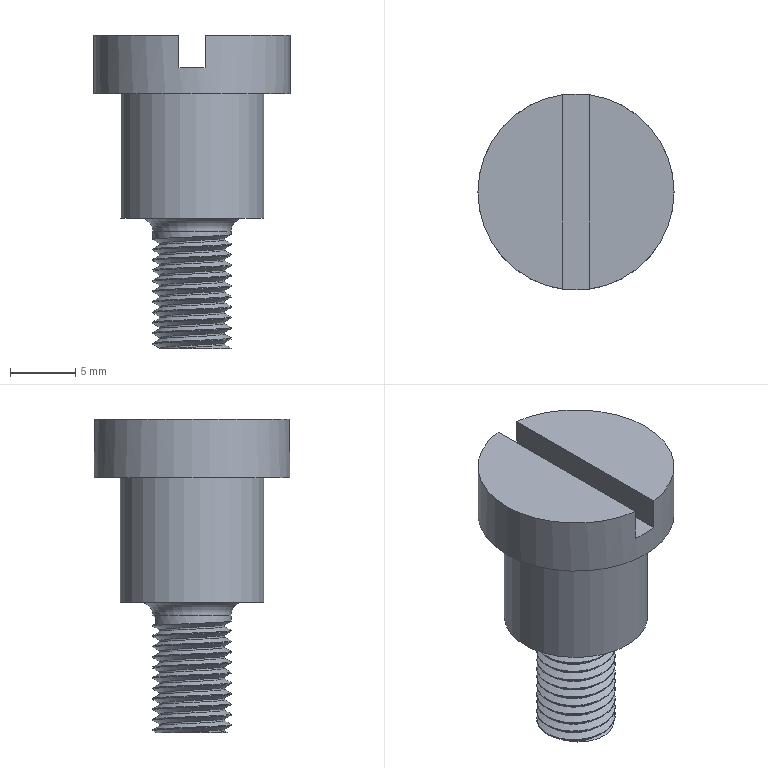Component | NX | LOCKING_SCREW | 1 solid | 16 faces | volume 1866 mm3 | plane 9 | cylinder 4 | spline 2 | torus 1 | commonest cylinder face diameters 15 x1 11 x1 6 x1 5 x1